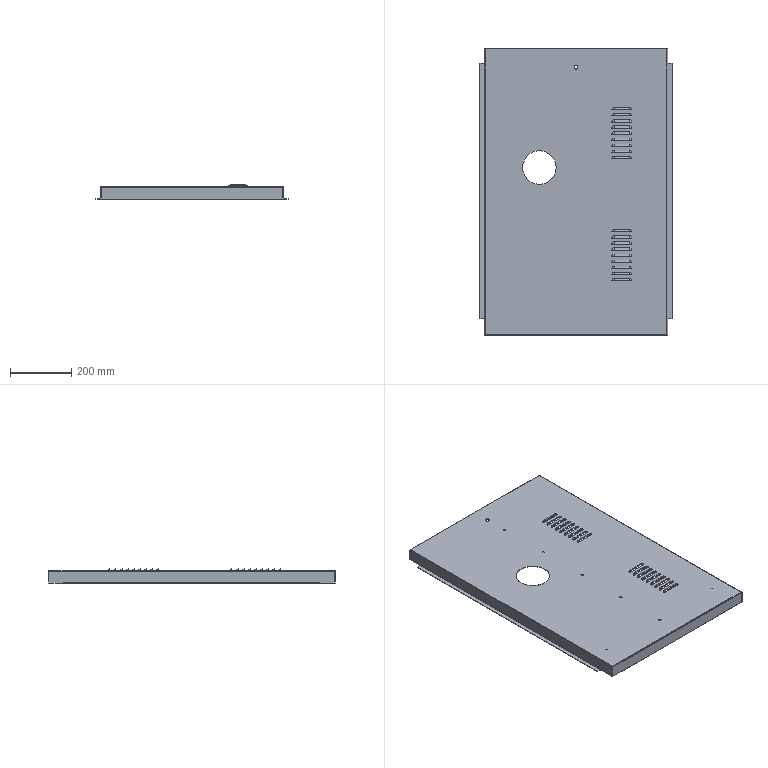Component | SolidWorks | RightSidePlate400AType40001100-2 | 1 solid | 342 faces | volume 1014851 mm3 | cylinder 100 | plane 98 | torus 72 | sphere 72 | commonest cylinder face diameters 4 x18 12 x18 1 x18 15 x18 8 x10 4.473 x5 1.473 x5 6 x4